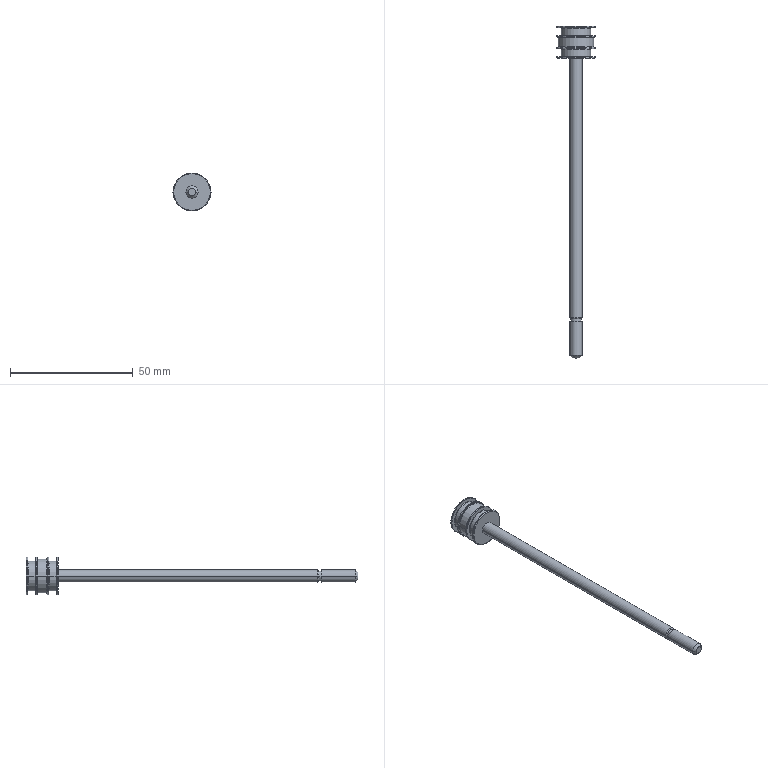Component | SolidWorks | PB_16x75_S_U_FA_M_2_0-1_16PB75URod-1 | 1 solid | 62 faces | box 15.5 x 135.36 x 15.5 mm | volume 4273 mm3 | cylinder 20 | torus 16 | cone 16 | plane 10 | commonest cylinder face diameters 15.5 x8 12 x4 5 x4 14.3 x2 4.38 x2
build123d program:
from build123d import *


with BuildPart() as part:
    # Sketch1 → Revolve1 (revolve)
    with BuildSketch(Plane.XY, mode=Mode.PRIVATE) as revolve1_sk:
        with BuildLine():
            Line((0, 0), (0, 1.45))
            Line((0, 1.45), (1.05, 2.5))
            Line((1.05, 2.5), (15, 2.5))
            Line((15, 2.5), (15, 2.19))
            Line((15, 2.19), (16, 2.19))
            Line((16, 2.19), (16.5, 2.5))
            Line((16.5, 2.5), (122.16, 2.5))
            Line((122.16, 2.5), (122.16, 7.45))
            ThreePointArc((122.16, 7.45), (122.248, 7.662), (122.46, 7.75))
            Line((122.46, 7.75), (122.76, 7.75))
            Line((122.76, 7.75), (122.86, 7.65))
            Line((122.86, 7.65), (122.86, 6.2))
            ThreePointArc((122.86, 6.2), (122.919, 6.059), (123.06, 6))
            Line((123.06, 6), (125.86, 6))
            ThreePointArc((125.86, 6), (126.001, 6.059), (126.06, 6.2))
            Line((126.06, 6.2), (126.06, 7.65))
            Line((126.06, 7.65), (126.16, 7.75))
            Line((126.16, 7.75), (126.56, 7.75))
            Line((126.56, 7.75), (126.66, 7.65))
            Line((126.66, 7.65), (126.66, 7.3))
            ThreePointArc((126.66, 7.3), (126.704, 7.194), (126.81, 7.15))
            Line((126.81, 7.15), (130.71, 7.15))
            ThreePointArc((130.71, 7.15), (130.816, 7.194), (130.86, 7.3))
            Line((130.86, 7.3), (130.86, 7.65))
            Line((130.86, 7.65), (130.96, 7.75))
            Line((130.96, 7.75), (131.36, 7.75))
            Line((131.36, 7.75), (131.46, 7.65))
            Line((131.46, 7.65), (131.46, 6.2))
            ThreePointArc((131.46, 6.2), (131.519, 6.059), (131.66, 6))
            Line((131.66, 6), (134.46, 6))
            ThreePointArc((134.46, 6), (134.601, 6.059), (134.66, 6.2))
            Line((134.66, 6.2), (134.66, 7.65))
            Line((134.66, 7.65), (134.76, 7.75))
            Line((134.76, 7.75), (135.06, 7.75))
            ThreePointArc((135.06, 7.75), (135.272, 7.662), (135.36, 7.45))
            Line((135.36, 7.45), (135.36, 0))
            Line((135.36, 0), (0, 0))
        make_face()
    revolve(revolve1_sk.sketch.rotate(Axis((135.36, 0, 0), (-1, 0, 0)), 270), axis=Axis((135.36, 0, 0), (-1, 0, 0)))


solid = part.part

# Placed as in the assembly
solid = solid.moved(Location((45, -250.5, 55), (0, 0, 90)))